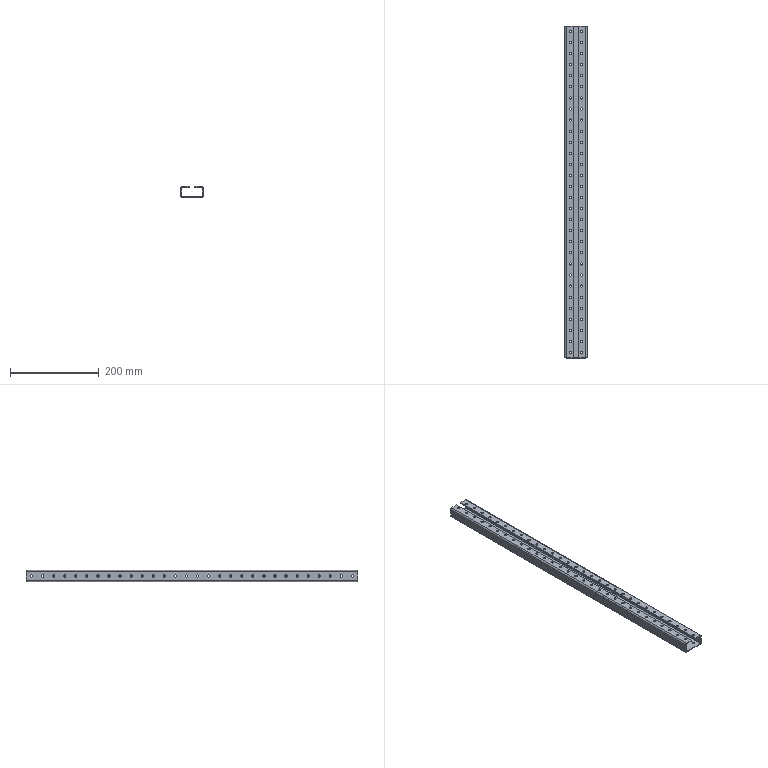Component | SolidWorks | Beam(No.10)-1 | 1 solid | 398 faces | volume 182031 mm3 | cylinder 368 | plane 30 | commonest cylinder face diameters 5 x360 6 x4 2 x4 | material Plain Carbon Steel